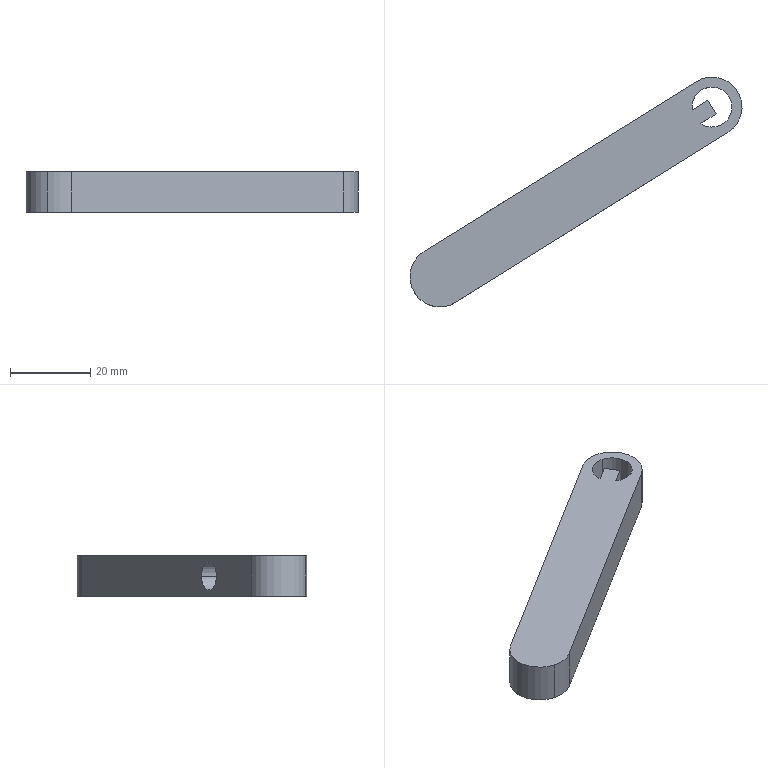Component | SolidWorks | FRocker-3 | 1 solid | 16 faces | box 82.86 x 57.36 x 10 mm | volume 12791 mm3 | cylinder 8 | plane 8 | commonest cylinder face diameters 10 x3 15 x3 7 x2
build123d program:
from build123d import *

# Parameters (mm, degrees)
BOSS_EXTRUDE1_DEPTH = 10
CUT_EXTRUDE1_DEPTH  = 10
SKETCH3_R           = 3.5
CUT_EXTRUDE2_DEPTH  = 10


with BuildPart() as part:
    # Sketch1 → Boss-Extrude1 (new body)
    with BuildSketch(Plane.XY):
        with BuildLine():
            Line((-210.677, 89.978), (-269.646, 35.916))
            ThreePointArc((-269.646, 35.916), (-280.242, 36.376), (-279.782, 46.973))
            Line((-279.782, 46.973), (-220.814, 101.035))
            ThreePointArc((-220.814, 101.035), (-210.217, 100.575), (-210.677, 89.978))
        make_face()
    extrude(amount=BOSS_EXTRUDE1_DEPTH)

    # Sketch2 → Cut-Extrude1 (cut)
    with BuildSketch(Plane(origin=(0, 0, 0), x_dir=(-1, 0, 0), z_dir=(0, 0, -1))):
        with BuildLine():
            Line((217.097, 96.981), (220.475, 93.884))
            ThreePointArc((220.475, 93.884), (220.678, 94.684), (220.746, 95.507))
            ThreePointArc((220.746, 95.507), (211.555, 98.233), (217.772, 90.936))
            Line((217.772, 90.936), (214.394, 94.033))
            Line((214.394, 94.033), (217.097, 96.981))
        make_face()
    extrude(amount=-CUT_EXTRUDE1_DEPTH, mode=Mode.SUBTRACT)

    # Sketch3 → Cut-Extrude2 (cut)
    with BuildSketch(Plane(origin=(-141.032, 153.83, 0), x_dir=(-0.7371, -0.6758, 0), z_dir=(0.6758, -0.7371, 0))):
        with Locations(Location((154.486, -5, 0), (0, 0, 180))):
            Circle(SKETCH3_R)
    extrude(amount=-CUT_EXTRUDE2_DEPTH, mode=Mode.SUBTRACT)


solid = part.part

# Placed as in the assembly
solid = solid.moved(Location((-254.541, 280.96, -27.818), (-180, 0, -74.488)))
STEP:
#1=CARTESIAN_POINT('',(-10.738,0.464,-1.292));
#2=VERTEX_POINT('',#1);
#3=CARTESIAN_POINT('',(-10.505,0.6099,-1.292));
#4=VERTEX_POINT('',#3);
#5=CARTESIAN_POINT('',(-10.621,0.537,-1.292));
#6=DIRECTION('',(-0.5295,0.8483,0.));
#7=DIRECTION('',(0.8483,0.5295,0.));
#8=AXIS2_PLACEMENT_3D('',#5,#6,#7);
#9=CIRCLE('',#8,0.1378);
#10=EDGE_CURVE('',#2,#4,#9,.T.);
#11=ORIENTED_EDGE('',*,*,#10,.F.);
#12=CARTESIAN_POINT('',(-10.947,0.798,-1.292));
#13=VERTEX_POINT('',#12);
#14=CARTESIAN_POINT('',(-10.738,0.464,-1.292));
#15=DIRECTION('',(-0.5295,0.8483,0.));
#16=VECTOR('',#15,39.37);
#17=LINE('',#14,#16);
#18=EDGE_CURVE('',#2,#13,#17,.T.);
#19=ORIENTED_EDGE('',*,*,#18,.T.);
#20=CARTESIAN_POINT('',(-10.713,0.9439,-1.292));
#21=VERTEX_POINT('',#20);
#22=CARTESIAN_POINT('',(-10.83,0.8709,-1.292));
#23=DIRECTION('',(-0.5295,0.8483,0.));
#24=DIRECTION('',(0.8483,0.5295,0.));
#25=AXIS2_PLACEMENT_3D('',#22,#23,#24);
#26=CIRCLE('',#25,0.1378);
#27=EDGE_CURVE('',#13,#21,#26,.T.);
#28=ORIENTED_EDGE('',*,*,#27,.T.);
#29=CARTESIAN_POINT('',(-10.505,0.6099,-1.292));
#30=DIRECTION('',(-0.5295,0.8483,0.));
#31=VECTOR('',#30,39.37);
#32=LINE('',#29,#31);
#33=EDGE_CURVE('',#4,#21,#32,.T.);
#34=ORIENTED_EDGE('',*,*,#33,.F.);
#35=EDGE_LOOP('',(#11,#19,#28,#34));
#36=FACE_OUTER_BOUND('',#35,.T.);
#37=CARTESIAN_POINT('',(-10.621,0.537,-1.292));
#38=DIRECTION('',(-0.5295,0.8483,0.));
#39=DIRECTION('',(0.8483,0.5295,0.));
#40=AXIS2_PLACEMENT_3D('',#37,#38,#39);
#41=CYLINDRICAL_SURFACE('',#40,0.1378);
#42=ADVANCED_FACE('',(#36),#41,.F.);
#43=CARTESIAN_POINT('',(-8.617,2.061,-1.489));
#44=VERTEX_POINT('',#43);
#45=CARTESIAN_POINT('',(-8.864,1.843,-1.489));
#46=VERTEX_POINT('',#45);
#47=CARTESIAN_POINT('',(-8.67,1.871,-1.489));
#48=DIRECTION('',(0.,-0.,1.));
#49=DIRECTION('',(-0.2674,-0.9636,0.));
#50=AXIS2_PLACEMENT_3D('',#47,#48,#49);
#51=CIRCLE('',#50,0.1969);
#52=EDGE_CURVE('',#44,#46,#51,.T.);
#53=ORIENTED_EDGE('',*,*,#52,.F.);
#54=CARTESIAN_POINT('',(-8.617,2.061,-1.095));
#55=VERTEX_POINT('',#54);
#56=CARTESIAN_POINT('',(-8.617,2.061,-1.489));
#57=DIRECTION('',(0.,-0.,1.));
#58=VECTOR('',#57,39.37);
#59=LINE('',#56,#58);
#60=EDGE_CURVE('',#44,#55,#59,.T.);
#61=ORIENTED_EDGE('',*,*,#60,.T.);
#62=CARTESIAN_POINT('',(-8.864,1.843,-1.095));
#63=VERTEX_POINT('',#62);
#64=CARTESIAN_POINT('',(-8.67,1.871,-1.095));
#65=DIRECTION('',(0.,-0.,1.));
#66=DIRECTION('',(-0.2674,-0.9636,0.));
#67=AXIS2_PLACEMENT_3D('',#64,#65,#66);
#68=CIRCLE('',#67,0.1969);
#69=EDGE_CURVE('',#55,#63,#68,.T.);
#70=ORIENTED_EDGE('',*,*,#69,.T.);
#71=CARTESIAN_POINT('',(-8.864,1.843,-1.489));
#72=DIRECTION('',(0.,-0.,1.));
#73=VECTOR('',#72,39.37);
#74=LINE('',#71,#73);
#75=EDGE_CURVE('',#46,#63,#74,.T.);
#76=ORIENTED_EDGE('',*,*,#75,.F.);
#77=EDGE_LOOP('',(#53,#61,#70,#76));
#78=FACE_OUTER_BOUND('',#77,.T.);
#79=CARTESIAN_POINT('',(-8.67,1.871,-1.489));
#80=DIRECTION('',(0.,-0.,1.));
#81=DIRECTION('',(-0.2674,-0.9636,0.));
#82=AXIS2_PLACEMENT_3D('',#79,#80,#81);
#83=CYLINDRICAL_SURFACE('',#82,0.1969);
#84=ADVANCED_FACE('',(#78),#83,.F.);
#85=ORIENTED_EDGE('',*,*,#60,.F.);
#86=CARTESIAN_POINT('',(-8.722,1.682,-1.489));
#87=VERTEX_POINT('',#86);
#88=CARTESIAN_POINT('',(-8.67,1.871,-1.489));
#89=DIRECTION('',(0.,-0.,1.));
#90=DIRECTION('',(-0.2674,-0.9636,0.));
#91=AXIS2_PLACEMENT_3D('',#88,#89,#90);
#92=CIRCLE('',#91,0.1969);
#93=EDGE_CURVE('',#87,#44,#92,.T.);
#94=ORIENTED_EDGE('',*,*,#93,.F.);
#95=CARTESIAN_POINT('',(-8.722,1.682,-1.095));
#96=VERTEX_POINT('',#95);
#97=CARTESIAN_POINT('',(-8.722,1.682,-1.489));
#98=DIRECTION('',(0.,-0.,1.));
#99=VECTOR('',#98,39.37);
#100=LINE('',#97,#99);
#101=EDGE_CURVE('',#87,#96,#100,.T.);
#102=ORIENTED_EDGE('',*,*,#101,.T.);
#103=CARTESIAN_POINT('',(-8.67,1.871,-1.095));
#104=DIRECTION('',(0.,-0.,1.));
#105=DIRECTION('',(-0.2674,-0.9636,0.));
#106=AXIS2_PLACEMENT_3D('',#103,#104,#105);
#107=CIRCLE('',#106,0.1969);
#108=EDGE_CURVE('',#96,#55,#107,.T.);
#109=ORIENTED_EDGE('',*,*,#108,.T.);
#110=EDGE_LOOP('',(#85,#94,#102,#109));
#111=FACE_OUTER_BOUND('',#110,.T.);
#112=CARTESIAN_POINT('',(-8.67,1.871,-1.489));
#113=DIRECTION('',(0.,-0.,1.));
#114=DIRECTION('',(-0.2674,-0.9636,0.));
#115=AXIS2_PLACEMENT_3D('',#112,#113,#114);
#116=CYLINDRICAL_SURFACE('',#115,0.1969);
#117=ADVANCED_FACE('',(#111),#116,.F.);
#118=CARTESIAN_POINT('',(-11.42,-0.08103,-1.489));
#119=VERTEX_POINT('',#118);
#120=CARTESIAN_POINT('',(-11.498,0.454,-1.489));
#121=VERTEX_POINT('',#120);
#122=CARTESIAN_POINT('',(-11.341,0.2035,-1.489));
#123=DIRECTION('',(-0.,0.,-1.));
#124=DIRECTION('',(0.2674,0.9636,0.));
#125=AXIS2_PLACEMENT_3D('',#122,#123,#124);
#126=CIRCLE('',#125,0.2953);
#127=EDGE_CURVE('',#119,#121,#126,.T.);
#128=ORIENTED_EDGE('',*,*,#127,.F.);
#129=CARTESIAN_POINT('',(-11.42,-0.08103,-1.095));
#130=VERTEX_POINT('',#129);
#131=CARTESIAN_POINT('',(-11.42,-0.08103,-1.489));
#132=DIRECTION('',(0.,-0.,1.));
#133=VECTOR('',#132,39.37);
#134=LINE('',#131,#133);
#135=EDGE_CURVE('',#119,#130,#134,.T.);
#136=ORIENTED_EDGE('',*,*,#135,.T.);
#137=CARTESIAN_POINT('',(-11.498,0.454,-1.095));
#138=VERTEX_POINT('',#137);
#139=CARTESIAN_POINT('',(-11.341,0.2035,-1.095));
#140=DIRECTION('',(-0.,0.,-1.));
#141=DIRECTION('',(0.2674,0.9636,0.));
#142=AXIS2_PLACEMENT_3D('',#139,#140,#141);
#143=CIRCLE('',#142,0.2953);
#144=EDGE_CURVE('',#130,#138,#143,.T.);
#145=ORIENTED_EDGE('',*,*,#144,.T.);
#146=CARTESIAN_POINT('',(-11.498,0.454,-1.489));
#147=DIRECTION('',(0.,-0.,1.));
#148=VECTOR('',#147,39.37);
#149=LINE('',#146,#148);
#150=EDGE_CURVE('',#121,#138,#149,.T.);
#151=ORIENTED_EDGE('',*,*,#150,.F.);
#152=EDGE_LOOP('',(#128,#136,#145,#151));
#153=FACE_OUTER_BOUND('',#152,.T.);
#154=CARTESIAN_POINT('',(-11.341,0.2035,-1.489));
#155=DIRECTION('',(0.,-0.,1.));
#156=DIRECTION('',(-0.2674,-0.9636,0.));
#157=AXIS2_PLACEMENT_3D('',#154,#155,#156);
#158=CYLINDRICAL_SURFACE('',#157,0.2953);
#159=ADVANCED_FACE('',(#153),#158,.T.);
#160=CARTESIAN_POINT('',(-8.513,1.621,-1.489));
#161=VERTEX_POINT('',#160);
#162=CARTESIAN_POINT('',(-11.185,-0.04699,-1.489));
#163=VERTEX_POINT('',#162);
#164=CARTESIAN_POINT('',(-5.358,3.591,-1.489));
#165=DIRECTION('',(-0.8483,-0.5295,0.));
#166=VECTOR('',#165,39.37);
#167=LINE('',#164,#166);
#168=EDGE_CURVE('',#161,#163,#167,.T.);
#169=ORIENTED_EDGE('',*,*,#168,.T.);
#170=CARTESIAN_POINT('',(-11.341,0.2035,-1.489));
#171=DIRECTION('',(-0.,0.,-1.));
#172=DIRECTION('',(0.2674,0.9636,0.));
#173=AXIS2_PLACEMENT_3D('',#170,#171,#172);
#174=CIRCLE('',#173,0.2953);
#175=EDGE_CURVE('',#163,#119,#174,.T.);
#176=ORIENTED_EDGE('',*,*,#175,.T.);
#177=ORIENTED_EDGE('',*,*,#127,.T.);
#178=CARTESIAN_POINT('',(-8.826,2.122,-1.489));
#179=VERTEX_POINT('',#178);
#180=CARTESIAN_POINT('',(-5.671,4.092,-1.489));
#181=DIRECTION('',(-0.8483,-0.5295,0.));
#182=VECTOR('',#181,39.37);
#183=LINE('',#180,#182);
#184=EDGE_CURVE('',#179,#121,#183,.T.);
#185=ORIENTED_EDGE('',*,*,#184,.F.);
#186=CARTESIAN_POINT('',(-8.67,1.871,-1.489));
#187=DIRECTION('',(-0.,0.,-1.));
#188=DIRECTION('',(0.2674,0.9636,0.));
#189=AXIS2_PLACEMENT_3D('',#186,#187,#188);
#190=CIRCLE('',#189,0.2953);
#191=EDGE_CURVE('',#179,#161,#190,.T.);
#192=ORIENTED_EDGE('',*,*,#191,.T.);
#193=EDGE_LOOP('',(#169,#176,#177,#185,#192));
#194=FACE_OUTER_BOUND('',#193,.T.);
#195=CARTESIAN_POINT('',(-8.628,1.805,-1.489));
#196=VERTEX_POINT('',#195);
#197=CARTESIAN_POINT('',(-8.711,1.938,-1.489));
#198=VERTEX_POINT('',#197);
#199=CARTESIAN_POINT('',(-13.177,9.092,-1.489));
#200=DIRECTION('',(-0.5295,0.8483,0.));
#201=VECTOR('',#200,39.37);
#202=LINE('',#199,#201);
#203=EDGE_CURVE('',#196,#198,#202,.T.);
#204=ORIENTED_EDGE('',*,*,#203,.F.);
#205=CARTESIAN_POINT('',(-8.781,1.709,-1.489));
#206=VERTEX_POINT('',#205);
#207=CARTESIAN_POINT('',(-5.472,3.774,-1.489));
#208=DIRECTION('',(0.8483,0.5295,-0.));
#209=VECTOR('',#208,39.37);
#210=LINE('',#207,#209);
#211=EDGE_CURVE('',#206,#196,#210,.T.);
#212=ORIENTED_EDGE('',*,*,#211,.F.);
#213=CARTESIAN_POINT('',(-8.67,1.871,-1.489));
#214=DIRECTION('',(0.,-0.,1.));
#215=DIRECTION('',(-0.2674,-0.9636,0.));
#216=AXIS2_PLACEMENT_3D('',#213,#214,#215);
#217=CIRCLE('',#216,0.1969);
#218=EDGE_CURVE('',#206,#87,#217,.T.);
#219=ORIENTED_EDGE('',*,*,#218,.T.);
#220=ORIENTED_EDGE('',*,*,#93,.T.);
#221=ORIENTED_EDGE('',*,*,#52,.T.);
#222=CARTESIAN_POINT('',(-5.556,3.908,-1.489));
#223=DIRECTION('',(0.8483,0.5295,-0.));
#224=VECTOR('',#223,39.37);
#225=LINE('',#222,#224);
#226=EDGE_CURVE('',#46,#198,#225,.T.);
#227=ORIENTED_EDGE('',*,*,#226,.T.);
#228=EDGE_LOOP('',(#204,#212,#219,#220,#221,#227));
#229=FACE_BOUND('',#228,.T.);
#230=CARTESIAN_POINT('',(-10.021,11.061,-1.489));
#231=DIRECTION('',(-0.,0.,-1.));
#232=DIRECTION('',(0.2674,0.9636,0.));
#233=AXIS2_PLACEMENT_3D('',#230,#231,#232);
#234=PLANE('',#233);
#235=ADVANCED_FACE('',(#194,#229),#234,.T.);
#236=CARTESIAN_POINT('',(-8.513,1.621,-1.095));
#237=VERTEX_POINT('',#236);
#238=CARTESIAN_POINT('',(-11.185,-0.04699,-1.095));
#239=VERTEX_POINT('',#238);
#240=CARTESIAN_POINT('',(-5.358,3.591,-1.095));
#241=DIRECTION('',(-0.8483,-0.5295,0.));
#242=VECTOR('',#241,39.37);
#243=LINE('',#240,#242);
#244=EDGE_CURVE('',#237,#239,#243,.T.);
#245=ORIENTED_EDGE('',*,*,#244,.F.);
#246=CARTESIAN_POINT('',(-8.826,2.122,-1.095));
#247=VERTEX_POINT('',#246);
#248=CARTESIAN_POINT('',(-8.67,1.871,-1.095));
#249=DIRECTION('',(-0.,0.,-1.));
#250=DIRECTION('',(0.2674,0.9636,0.));
#251=AXIS2_PLACEMENT_3D('',#248,#249,#250);
#252=CIRCLE('',#251,0.2953);
#253=EDGE_CURVE('',#247,#237,#252,.T.);
#254=ORIENTED_EDGE('',*,*,#253,.F.);
#255=CARTESIAN_POINT('',(-5.671,4.092,-1.095));
#256=DIRECTION('',(-0.8483,-0.5295,0.));
#257=VECTOR('',#256,39.37);
#258=LINE('',#255,#257);
#259=EDGE_CURVE('',#247,#138,#258,.T.);
#260=ORIENTED_EDGE('',*,*,#259,.T.);
#261=ORIENTED_EDGE('',*,*,#144,.F.);
#262=CARTESIAN_POINT('',(-11.341,0.2035,-1.095));
#263=DIRECTION('',(-0.,0.,-1.));
#264=DIRECTION('',(0.2674,0.9636,0.));
#265=AXIS2_PLACEMENT_3D('',#262,#263,#264);
#266=CIRCLE('',#265,0.2953);
#267=EDGE_CURVE('',#239,#130,#266,.T.);
#268=ORIENTED_EDGE('',*,*,#267,.F.);
#269=EDGE_LOOP('',(#245,#254,#260,#261,#268));
#270=FACE_OUTER_BOUND('',#269,.T.);
#271=CARTESIAN_POINT('',(-8.781,1.709,-1.095));
#272=VERTEX_POINT('',#271);
#273=CARTESIAN_POINT('',(-8.628,1.805,-1.095));
#274=VERTEX_POINT('',#273);
#275=CARTESIAN_POINT('',(-5.472,3.774,-1.095));
#276=DIRECTION('',(0.8483,0.5295,-0.));
#277=VECTOR('',#276,39.37);
#278=LINE('',#275,#277);
#279=EDGE_CURVE('',#272,#274,#278,.T.);
#280=ORIENTED_EDGE('',*,*,#279,.T.);
#281=CARTESIAN_POINT('',(-8.711,1.938,-1.095));
#282=VERTEX_POINT('',#281);
#283=CARTESIAN_POINT('',(-13.177,9.092,-1.095));
#284=DIRECTION('',(-0.5295,0.8483,0.));
#285=VECTOR('',#284,39.37);
#286=LINE('',#283,#285);
#287=EDGE_CURVE('',#274,#282,#286,.T.);
#288=ORIENTED_EDGE('',*,*,#287,.T.);
#289=CARTESIAN_POINT('',(-5.556,3.908,-1.095));
#290=DIRECTION('',(0.8483,0.5295,-0.));
#291=VECTOR('',#290,39.37);
#292=LINE('',#289,#291);
#293=EDGE_CURVE('',#63,#282,#292,.T.);
#294=ORIENTED_EDGE('',*,*,#293,.F.);
#295=ORIENTED_EDGE('',*,*,#69,.F.);
#296=ORIENTED_EDGE('',*,*,#108,.F.);
#297=CARTESIAN_POINT('',(-8.67,1.871,-1.095));
#298=DIRECTION('',(0.,-0.,1.));
#299=DIRECTION('',(-0.2674,-0.9636,0.));
#300=AXIS2_PLACEMENT_3D('',#297,#298,#299);
#301=CIRCLE('',#300,0.1969);
#302=EDGE_CURVE('',#272,#96,#301,.T.);
#303=ORIENTED_EDGE('',*,*,#302,.F.);
#304=EDGE_LOOP('',(#280,#288,#294,#295,#296,#303));
#305=FACE_BOUND('',#304,.T.);
#306=CARTESIAN_POINT('',(-10.021,11.061,-1.095));
#307=DIRECTION('',(-0.,0.,-1.));
#308=DIRECTION('',(0.2674,0.9636,0.));
#309=AXIS2_PLACEMENT_3D('',#306,#307,#308);
#310=PLANE('',#309);
#311=ADVANCED_FACE('',(#270,#305),#310,.F.);
#312=ORIENTED_EDGE('',*,*,#244,.T.);
#313=CARTESIAN_POINT('',(-11.185,-0.04699,-1.489));
#314=DIRECTION('',(0.,-0.,1.));
#315=VECTOR('',#314,39.37);
#316=LINE('',#313,#315);
#317=EDGE_CURVE('',#163,#239,#316,.T.);
#318=ORIENTED_EDGE('',*,*,#317,.F.);
#319=ORIENTED_EDGE('',*,*,#168,.F.);
#320=CARTESIAN_POINT('',(-8.513,1.621,-1.489));
#321=DIRECTION('',(0.,-0.,1.));
#322=VECTOR('',#321,39.37);
#323=LINE('',#320,#322);
#324=EDGE_CURVE('',#161,#237,#323,.T.);
#325=ORIENTED_EDGE('',*,*,#324,.T.);
#326=EDGE_LOOP('',(#312,#318,#319,#325));
#327=FACE_OUTER_BOUND('',#326,.T.);
#328=CARTESIAN_POINT('',(-5.358,3.591,-1.489));
#329=DIRECTION('',(-0.5295,0.8483,0.));
#330=DIRECTION('',(0.8483,0.5295,-0.));
#331=AXIS2_PLACEMENT_3D('',#328,#329,#330);
#332=PLANE('',#331);
#333=ADVANCED_FACE('',(#327),#332,.F.);
#334=ORIENTED_EDGE('',*,*,#135,.F.);
#335=ORIENTED_EDGE('',*,*,#175,.F.);
#336=ORIENTED_EDGE('',*,*,#317,.T.);
#337=ORIENTED_EDGE('',*,*,#267,.T.);
#338=EDGE_LOOP('',(#334,#335,#336,#337));
#339=FACE_OUTER_BOUND('',#338,.T.);
#340=CARTESIAN_POINT('',(-11.341,0.2035,-1.489));
#341=DIRECTION('',(0.,-0.,1.));
#342=DIRECTION('',(-0.2674,-0.9636,0.));
#343=AXIS2_PLACEMENT_3D('',#340,#341,#342);
#344=CYLINDRICAL_SURFACE('',#343,0.2953);
#345=ADVANCED_FACE('',(#339),#344,.T.);
#346=CARTESIAN_POINT('',(-10.83,0.8709,-1.292));
#347=DIRECTION('',(-0.5295,0.8483,0.));
#348=DIRECTION('',(0.8483,0.5295,0.));
#349=AXIS2_PLACEMENT_3D('',#346,#347,#348);
#350=CIRCLE('',#349,0.1378);
#351=EDGE_CURVE('',#21,#13,#350,.T.);
#352=ORIENTED_EDGE('',*,*,#351,.F.);
#353=ORIENTED_EDGE('',*,*,#27,.F.);
#354=EDGE_LOOP('',(#352,#353));
#355=FACE_BOUND('',#354,.T.);
#356=ORIENTED_EDGE('',*,*,#259,.F.);
#357=CARTESIAN_POINT('',(-8.826,2.122,-1.489));
#358=DIRECTION('',(0.,-0.,1.));
#359=VECTOR('',#358,39.37);
#360=LINE('',#357,#359);
#361=EDGE_CURVE('',#179,#247,#360,.T.);
#362=ORIENTED_EDGE('',*,*,#361,.F.);
#363=ORIENTED_EDGE('',*,*,#184,.T.);
#364=ORIENTED_EDGE('',*,*,#150,.T.);
#365=EDGE_LOOP('',(#356,#362,#363,#364));
#366=FACE_OUTER_BOUND('',#365,.T.);
#367=CARTESIAN_POINT('',(-5.671,4.092,-1.489));
#368=DIRECTION('',(-0.5295,0.8483,0.));
#369=DIRECTION('',(0.8483,0.5295,-0.));
#370=AXIS2_PLACEMENT_3D('',#367,#368,#369);
#371=PLANE('',#370);
#372=ADVANCED_FACE('',(#355,#366),#371,.T.);
#373=ORIENTED_EDGE('',*,*,#253,.T.);
#374=ORIENTED_EDGE('',*,*,#324,.F.);
#375=ORIENTED_EDGE('',*,*,#191,.F.);
#376=ORIENTED_EDGE('',*,*,#361,.T.);
#377=EDGE_LOOP('',(#373,#374,#375,#376));
#378=FACE_OUTER_BOUND('',#377,.T.);
#379=CARTESIAN_POINT('',(-8.67,1.871,-1.489));
#380=DIRECTION('',(0.,-0.,1.));
#381=DIRECTION('',(-0.2674,-0.9636,0.));
#382=AXIS2_PLACEMENT_3D('',#379,#380,#381);
#383=CYLINDRICAL_SURFACE('',#382,0.2953);
#384=ADVANCED_FACE('',(#378),#383,.T.);
#385=ORIENTED_EDGE('',*,*,#279,.F.);
#386=CARTESIAN_POINT('',(-8.781,1.709,-1.489));
#387=DIRECTION('',(0.,-0.,1.));
#388=VECTOR('',#387,39.37);
#389=LINE('',#386,#388);
#390=EDGE_CURVE('',#206,#272,#389,.T.);
#391=ORIENTED_EDGE('',*,*,#390,.F.);
#392=ORIENTED_EDGE('',*,*,#211,.T.);
#393=CARTESIAN_POINT('',(-8.628,1.805,-1.489));
#394=DIRECTION('',(0.,-0.,1.));
#395=VECTOR('',#394,39.37);
#396=LINE('',#393,#395);
#397=EDGE_CURVE('',#196,#274,#396,.T.);
#398=ORIENTED_EDGE('',*,*,#397,.T.);
#399=EDGE_LOOP('',(#385,#391,#392,#398));
#400=FACE_OUTER_BOUND('',#399,.T.);
#401=CARTESIAN_POINT('',(-5.472,3.774,-1.489));
#402=DIRECTION('',(0.5295,-0.8483,-0.));
#403=DIRECTION('',(-0.8483,-0.5295,0.));
#404=AXIS2_PLACEMENT_3D('',#401,#402,#403);
#405=PLANE('',#404);
#406=ADVANCED_FACE('',(#400),#405,.T.);
#407=ORIENTED_EDGE('',*,*,#287,.F.);
#408=ORIENTED_EDGE('',*,*,#397,.F.);
#409=ORIENTED_EDGE('',*,*,#203,.T.);
#410=CARTESIAN_POINT('',(-8.711,1.938,-1.489));
#411=DIRECTION('',(0.,-0.,1.));
#412=VECTOR('',#411,39.37);
#413=LINE('',#410,#412);
#414=EDGE_CURVE('',#198,#282,#413,.T.);
#415=ORIENTED_EDGE('',*,*,#414,.T.);
#416=EDGE_LOOP('',(#407,#408,#409,#415));
#417=FACE_OUTER_BOUND('',#416,.T.);
#418=CARTESIAN_POINT('',(-13.177,9.092,-1.489));
#419=DIRECTION('',(0.8483,0.5295,-0.));
#420=DIRECTION('',(0.5295,-0.8483,-0.));
#421=AXIS2_PLACEMENT_3D('',#418,#419,#420);
#422=PLANE('',#421);
#423=ADVANCED_FACE('',(#417),#422,.T.);
#424=ORIENTED_EDGE('',*,*,#293,.T.);
#425=ORIENTED_EDGE('',*,*,#414,.F.);
#426=ORIENTED_EDGE('',*,*,#226,.F.);
#427=ORIENTED_EDGE('',*,*,#75,.T.);
#428=EDGE_LOOP('',(#424,#425,#426,#427));
#429=FACE_OUTER_BOUND('',#428,.T.);
#430=CARTESIAN_POINT('',(-5.556,3.908,-1.489));
#431=DIRECTION('',(0.5295,-0.8483,-0.));
#432=DIRECTION('',(-0.8483,-0.5295,0.));
#433=AXIS2_PLACEMENT_3D('',#430,#431,#432);
#434=PLANE('',#433);
#435=ADVANCED_FACE('',(#429),#434,.F.);
#436=ORIENTED_EDGE('',*,*,#101,.F.);
#437=ORIENTED_EDGE('',*,*,#218,.F.);
#438=ORIENTED_EDGE('',*,*,#390,.T.);
#439=ORIENTED_EDGE('',*,*,#302,.T.);
#440=EDGE_LOOP('',(#436,#437,#438,#439));
#441=FACE_OUTER_BOUND('',#440,.T.);
#442=CARTESIAN_POINT('',(-8.67,1.871,-1.489));
#443=DIRECTION('',(0.,-0.,1.));
#444=DIRECTION('',(-0.2674,-0.9636,0.));
#445=AXIS2_PLACEMENT_3D('',#442,#443,#444);
#446=CYLINDRICAL_SURFACE('',#445,0.1969);
#447=ADVANCED_FACE('',(#441),#446,.F.);
#448=ORIENTED_EDGE('',*,*,#18,.F.);
#449=CARTESIAN_POINT('',(-10.621,0.537,-1.292));
#450=DIRECTION('',(-0.5295,0.8483,0.));
#451=DIRECTION('',(0.8483,0.5295,0.));
#452=AXIS2_PLACEMENT_3D('',#449,#450,#451);
#453=CIRCLE('',#452,0.1378);
#454=EDGE_CURVE('',#4,#2,#453,.T.);
#455=ORIENTED_EDGE('',*,*,#454,.F.);
#456=ORIENTED_EDGE('',*,*,#33,.T.);
#457=ORIENTED_EDGE('',*,*,#351,.T.);
#458=EDGE_LOOP('',(#448,#455,#456,#457));
#459=FACE_OUTER_BOUND('',#458,.T.);
#460=CARTESIAN_POINT('',(-10.621,0.537,-1.292));
#461=DIRECTION('',(-0.5295,0.8483,0.));
#462=DIRECTION('',(0.8483,0.5295,0.));
#463=AXIS2_PLACEMENT_3D('',#460,#461,#462);
#464=CYLINDRICAL_SURFACE('',#463,0.1378);
#465=ADVANCED_FACE('',(#459),#464,.F.);
#466=ORIENTED_EDGE('',*,*,#454,.T.);
#467=ORIENTED_EDGE('',*,*,#10,.T.);
#468=EDGE_LOOP('',(#466,#467));
#469=FACE_OUTER_BOUND('',#468,.T.);
#470=CARTESIAN_POINT('',(-5.462,3.758,-1.095));
#471=DIRECTION('',(-0.5295,0.8483,0.));
#472=DIRECTION('',(0.8483,0.5295,-0.));
#473=AXIS2_PLACEMENT_3D('',#470,#471,#472);
#474=PLANE('',#473);
#475=ADVANCED_FACE('',(#469),#474,.T.);
#476=CLOSED_SHELL('',(#42,#84,#117,#159,#235,#311,#333,#345,#372,#384,#406,#423,#435,#447,#465,#475));
#477=MANIFOLD_SOLID_BREP('',#476);
#478=CARTESIAN_POINT('',(0.,0.,0.));
#479=DIRECTION('',(0.,0.,1.));
#480=DIRECTION('',(1.,0.,0.));
#481=AXIS2_PLACEMENT_3D('',#478,#479,#480);
#482=(LENGTH_UNIT()NAMED_UNIT(*)SI_UNIT($,.METRE.));
#483=LENGTH_MEASURE_WITH_UNIT(LENGTH_MEASURE(0.0254),#482);
#484=DIMENSIONAL_EXPONENTS(1.,0.,0.,0.,0.,0.,0.);
#485=(CONVERSION_BASED_UNIT('',#483)LENGTH_UNIT()NAMED_UNIT(#484));
#486=UNCERTAINTY_MEASURE_WITH_UNIT(LENGTH_MEASURE(0.00001),#485,'','');
#487=(NAMED_UNIT(*)PLANE_ANGLE_UNIT()SI_UNIT($,.RADIAN.));
#488=(NAMED_UNIT(*)SI_UNIT($,.STERADIAN.)SOLID_ANGLE_UNIT());
#489=(GEOMETRIC_REPRESENTATION_CONTEXT(3)GLOBAL_UNCERTAINTY_ASSIGNED_CONTEXT((#486))GLOBAL_UNIT_ASSIGNED_CONTEXT((#485,#487,#488))REPRESENTATION_CONTEXT('',''));
#490=ADVANCED_BREP_SHAPE_REPRESENTATION('',(#477,#481),#489);
#491=COLOUR_RGB('',0.7922,0.8196,0.9333);
#492=FILL_AREA_STYLE_COLOUR('',#491);
#493=FILL_AREA_STYLE('',(#492));
#494=SURFACE_STYLE_FILL_AREA(#493);
#495=SURFACE_SIDE_STYLE('',(#494));
#496=SURFACE_STYLE_USAGE(.BOTH.,#495);
#497=PRESENTATION_STYLE_ASSIGNMENT((#496));
#498=STYLED_ITEM('',(#497),#477);
#499=PRESENTATION_LAYER_ASSIGNMENT('','',(#498));
#500=(LENGTH_UNIT()NAMED_UNIT(*)SI_UNIT($,.METRE.));
#501=LENGTH_MEASURE_WITH_UNIT(LENGTH_MEASURE(0.0254),#500);
#502=DIMENSIONAL_EXPONENTS(1.,0.,0.,0.,0.,0.,0.);
#503=(CONVERSION_BASED_UNIT('',#501)LENGTH_UNIT()NAMED_UNIT(#502));
#504=UNCERTAINTY_MEASURE_WITH_UNIT(LENGTH_MEASURE(0.00001),#503,'','');
#505=(NAMED_UNIT(*)PLANE_ANGLE_UNIT()SI_UNIT($,.RADIAN.));
#506=(NAMED_UNIT(*)SI_UNIT($,.STERADIAN.)SOLID_ANGLE_UNIT());
#507=(GEOMETRIC_REPRESENTATION_CONTEXT(3)GLOBAL_UNCERTAINTY_ASSIGNED_CONTEXT((#504))GLOBAL_UNIT_ASSIGNED_CONTEXT((#503,#505,#506))REPRESENTATION_CONTEXT('',''));
#508=MECHANICAL_DESIGN_GEOMETRIC_PRESENTATION_REPRESENTATION('',(#498),#507);